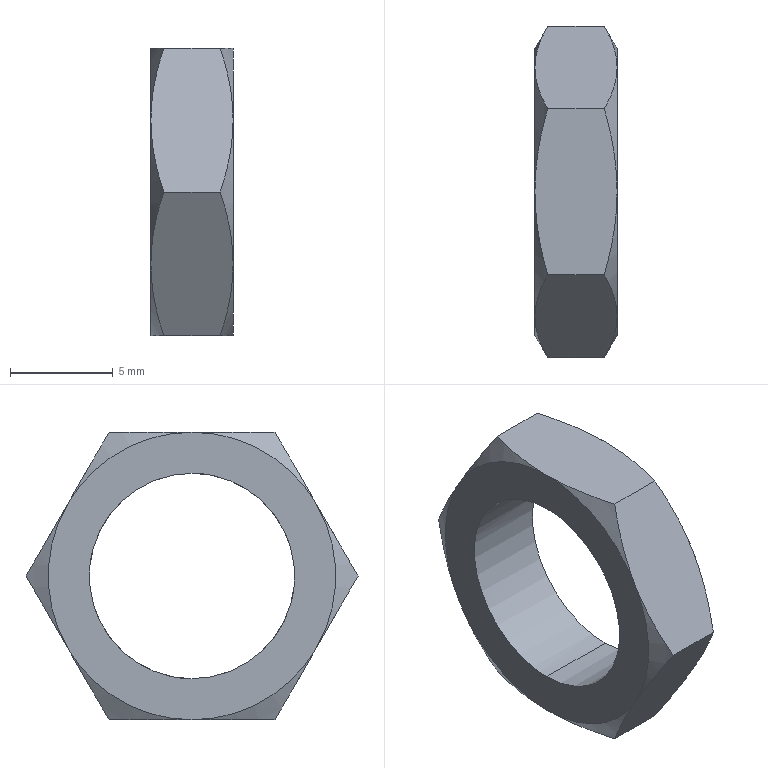Component | SolidWorks | 17268PB16x60SU(58)+(CS1-M-2)-1_1726816nut-1 | 1 solid | 22 faces | box 4 x 16.17 x 14 mm | volume 359 mm3 | cone 12 | plane 8 | cylinder 2 | commonest cylinder face diameters 10 x2
build123d program:
from build123d import *

# Parameters (mm, degrees)
CUT_EXTRUDE1_DEPTH               = 2
CUT_EXTRUDE1_DEPTH_BACK          = 2
SKETCH3_W                        = 28
SKETCH3_H                        = 28
THREAD_FIT_RELIEF_M10_DEPTH      = 12.416
THREAD_FIT_RELIEF_M10_DEPTH_BACK = 12.416
SKETCH1_R                        = 5


with BuildPart() as part:
    # Sketch1_2 → Revolve1 (revolve)
    with BuildSketch(Plane.XY, mode=Mode.PRIVATE) as revolve1_sk:
        Polygon((-2, 0), (-2, 7), (-1.192, 8.4), (1.192, 8.4), (2, 7), (2, 0), align=None)
    revolve(revolve1_sk.sketch.rotate(Axis((2, 0, 0), (-1, 0, 0)), 270), axis=Axis((2, 0, 0), (-1, 0, 0)))

    # Sketch2 → Cut-Revolve1 (revolve, cut)
    with BuildSketch(Plane.XY, mode=Mode.PRIVATE) as cut_revolve1_sk:
        Polygon((-2, 0), (-2, 5), (-1.188, 4.188), (1.188, 4.188), (2, 5), (2, 0), align=None)
    revolve(cut_revolve1_sk.sketch.rotate(Axis((2, 0, 0), (-1, 0, 0)), 270), axis=Axis((2, 0, 0), (-1, 0, 0)), mode=Mode.SUBTRACT)

    # Sketch3 → Cut-Extrude1 (cut, two sides: drawn at the far end of the back side and taken through both)
    with BuildSketch(Plane(origin=(0, 0, 0), x_dir=(0, 0, -1), z_dir=(1, 0, 0)).offset(-CUT_EXTRUDE1_DEPTH_BACK)):
        Rectangle(SKETCH3_W, SKETCH3_H)
        Polygon((-7, -4.041), (0, -8.083), (7, -4.041), (7, 4.041), (0, 8.083), (-7, 4.041), align=None, mode=Mode.SUBTRACT)
    extrude(amount=CUT_EXTRUDE1_DEPTH + CUT_EXTRUDE1_DEPTH_BACK, mode=Mode.SUBTRACT)

    # Sketch1 → Thread fit relief M10 (cut, two sides: drawn at the far end of the back side and taken through both)
    with BuildSketch(Plane.ZY.offset(2).offset(-THREAD_FIT_RELIEF_M10_DEPTH_BACK)):
        Circle(SKETCH1_R)
    extrude(amount=THREAD_FIT_RELIEF_M10_DEPTH + THREAD_FIT_RELIEF_M10_DEPTH_BACK, mode=Mode.SUBTRACT)


solid = part.part

# Placed as in the assembly
solid = solid.moved(Location((-73, -27.579, 21.5), (0, 0, 0)))
STEP:
#1=COLOUR_RGB('',0.7922,0.8196,0.9333);
#2=FILL_AREA_STYLE_COLOUR('',#1);
#3=FILL_AREA_STYLE('',(#2));
#4=SURFACE_STYLE_FILL_AREA(#3);
#5=SURFACE_SIDE_STYLE('',(#4));
#6=SURFACE_STYLE_USAGE(.BOTH.,#5);
#7=PRESENTATION_STYLE_ASSIGNMENT((#6));
#8=CARTESIAN_POINT('',(-2.795,-1.086,1.043));
#9=VERTEX_POINT('',#8);
#10=CARTESIAN_POINT('',(-2.795,-1.086,0.6496));
#11=VERTEX_POINT('',#10);
#12=CARTESIAN_POINT('',(-2.795,-1.086,0.8465));
#13=DIRECTION('',(-1.,0.,0.));
#14=DIRECTION('',(0.,0.,-1.));
#15=AXIS2_PLACEMENT_3D('',#12,#13,#14);
#16=CIRCLE('',#15,0.1969);
#17=EDGE_CURVE('',#9,#11,#16,.T.);
#18=ORIENTED_EDGE('',*,*,#17,.F.);
#19=CARTESIAN_POINT('',(-2.953,-1.086,1.043));
#20=VERTEX_POINT('',#19);
#21=CARTESIAN_POINT('',(-2.795,-1.086,1.043));
#22=DIRECTION('',(-1.,0.,0.));
#23=VECTOR('',#22,39.37);
#24=LINE('',#21,#23);
#25=EDGE_CURVE('',#9,#20,#24,.T.);
#26=ORIENTED_EDGE('',*,*,#25,.T.);
#27=CARTESIAN_POINT('',(-2.953,-1.086,0.6496));
#28=VERTEX_POINT('',#27);
#29=CARTESIAN_POINT('',(-2.953,-1.086,1.043));
#30=CARTESIAN_POINT('',(-2.953,-1.06,1.043));
#31=CARTESIAN_POINT('',(-2.953,-1.034,1.038));
#32=CARTESIAN_POINT('',(-2.953,-0.9867,1.018));
#33=CARTESIAN_POINT('',(-2.953,-0.9648,1.004));
#34=CARTESIAN_POINT('',(-2.953,-0.9284,0.9674));
#35=CARTESIAN_POINT('',(-2.953,-0.9138,0.9456));
#36=CARTESIAN_POINT('',(-2.953,-0.8941,0.898));
#37=CARTESIAN_POINT('',(-2.953,-0.8889,0.8722));
#38=CARTESIAN_POINT('',(-2.953,-0.8889,0.8207));
#39=CARTESIAN_POINT('',(-2.953,-0.8941,0.7949));
#40=CARTESIAN_POINT('',(-2.953,-0.9138,0.7473));
#41=CARTESIAN_POINT('',(-2.953,-0.9284,0.7255));
#42=CARTESIAN_POINT('',(-2.953,-0.9648,0.689));
#43=CARTESIAN_POINT('',(-2.953,-0.9867,0.6745));
#44=CARTESIAN_POINT('',(-2.953,-1.034,0.6547));
#45=CARTESIAN_POINT('',(-2.953,-1.06,0.6496));
#46=CARTESIAN_POINT('',(-2.953,-1.086,0.6496));
#47=B_SPLINE_CURVE_WITH_KNOTS('',3,(#29,#30,#31,#32,#33,#34,#35,#36,#37,#38,#39,#40,#41,#42,#43,#44,#45,#46),.UNSPECIFIED.,.F.,.F.,(4,2,2,2,2,2,2,2,4),(0.5,0.5625,0.625,0.6875,0.75,0.8125,0.875,0.9375,1.),.UNSPECIFIED.);
#48=EDGE_CURVE('',#20,#28,#47,.T.);
#49=ORIENTED_EDGE('',*,*,#48,.T.);
#50=CARTESIAN_POINT('',(-2.795,-1.086,0.6496));
#51=DIRECTION('',(-1.,0.,0.));
#52=VECTOR('',#51,39.37);
#53=LINE('',#50,#52);
#54=EDGE_CURVE('',#11,#28,#53,.T.);
#55=ORIENTED_EDGE('',*,*,#54,.F.);
#56=EDGE_LOOP('',(#18,#26,#49,#55));
#57=FACE_OUTER_BOUND('',#56,.T.);
#58=CARTESIAN_POINT('',(-2.795,-1.086,0.8465));
#59=DIRECTION('',(-1.,0.,0.));
#60=DIRECTION('',(0.,0.,-1.));
#61=AXIS2_PLACEMENT_3D('',#58,#59,#60);
#62=CYLINDRICAL_SURFACE('',#61,0.1969);
#63=ADVANCED_FACE('',(#57),#62,.F.);
#64=CARTESIAN_POINT('',(-2.928,-1.245,1.122));
#65=VERTEX_POINT('',#64);
#66=CARTESIAN_POINT('',(-2.953,-1.324,0.9843));
#67=VERTEX_POINT('',#66);
#68=CARTESIAN_POINT('',(-2.928,-1.245,1.122));
#69=CARTESIAN_POINT('',(-2.936,-1.258,1.1));
#70=CARTESIAN_POINT('',(-2.942,-1.271,1.077));
#71=CARTESIAN_POINT('',(-2.95,-1.298,1.031));
#72=CARTESIAN_POINT('',(-2.953,-1.311,1.008));
#73=CARTESIAN_POINT('',(-2.953,-1.324,0.9843));
#74=B_SPLINE_CURVE_WITH_KNOTS('',3,(#68,#69,#70,#71,#72,#73),.UNSPECIFIED.,.F.,.F.,(4,2,4),(0.00000024,0.002045,0.00409),.UNSPECIFIED.);
#75=EDGE_CURVE('',#65,#67,#74,.T.);
#76=ORIENTED_EDGE('',*,*,#75,.F.);
#77=CARTESIAN_POINT('',(-2.953,-1.086,1.122));
#78=VERTEX_POINT('',#77);
#79=CARTESIAN_POINT('',(-2.953,-1.086,1.122));
#80=CARTESIAN_POINT('',(-2.953,-1.113,1.122));
#81=CARTESIAN_POINT('',(-2.95,-1.14,1.122));
#82=CARTESIAN_POINT('',(-2.942,-1.193,1.122));
#83=CARTESIAN_POINT('',(-2.936,-1.219,1.122));
#84=CARTESIAN_POINT('',(-2.928,-1.245,1.122));
#85=B_SPLINE_CURVE_WITH_KNOTS('',3,(#79,#80,#81,#82,#83,#84),.UNSPECIFIED.,.F.,.F.,(4,2,4),(0.01133,0.01337,0.01542),.UNSPECIFIED.);
#86=EDGE_CURVE('',#78,#65,#85,.T.);
#87=ORIENTED_EDGE('',*,*,#86,.F.);
#88=CARTESIAN_POINT('',(-2.953,-1.086,0.8465));
#89=DIRECTION('',(-1.,0.,0.));
#90=DIRECTION('',(0.,0.,-1.));
#91=AXIS2_PLACEMENT_3D('',#88,#89,#90);
#92=CIRCLE('',#91,0.2756);
#93=EDGE_CURVE('',#67,#78,#92,.T.);
#94=ORIENTED_EDGE('',*,*,#93,.F.);
#95=EDGE_LOOP('',(#76,#87,#94));
#96=FACE_OUTER_BOUND('',#95,.T.);
#97=CARTESIAN_POINT('',(-2.921,-1.086,0.8465));
#98=DIRECTION('',(1.,-0.,-0.));
#99=DIRECTION('',(0.,0.,1.));
#100=AXIS2_PLACEMENT_3D('',#97,#98,#99);
#101=CONICAL_SURFACE('',#100,0.3307,1.047);
#102=ADVANCED_FACE('',(#96),#101,.T.);
#103=CARTESIAN_POINT('',(-2.928,-1.404,0.8465));
#104=VERTEX_POINT('',#103);
#105=CARTESIAN_POINT('',(-2.953,-1.324,0.9843));
#106=CARTESIAN_POINT('',(-2.953,-1.331,0.9726));
#107=CARTESIAN_POINT('',(-2.952,-1.338,0.9608));
#108=CARTESIAN_POINT('',(-2.95,-1.351,0.9376));
#109=CARTESIAN_POINT('',(-2.948,-1.358,0.926));
#110=CARTESIAN_POINT('',(-2.942,-1.378,0.8916));
#111=CARTESIAN_POINT('',(-2.936,-1.391,0.8689));
#112=CARTESIAN_POINT('',(-2.928,-1.404,0.8465));
#113=B_SPLINE_CURVE_WITH_KNOTS('',3,(#105,#106,#107,#108,#109,#110,#111,#112),.UNSPECIFIED.,.F.,.F.,(4,2,2,4),(0.00409,0.005108,0.006127,0.008164),.UNSPECIFIED.);
#114=EDGE_CURVE('',#67,#104,#113,.T.);
#115=ORIENTED_EDGE('',*,*,#114,.F.);
#116=CARTESIAN_POINT('',(-2.953,-1.324,0.7087));
#117=VERTEX_POINT('',#116);
#118=CARTESIAN_POINT('',(-2.953,-1.086,0.8465));
#119=DIRECTION('',(-1.,0.,0.));
#120=DIRECTION('',(0.,0.,-1.));
#121=AXIS2_PLACEMENT_3D('',#118,#119,#120);
#122=CIRCLE('',#121,0.2756);
#123=EDGE_CURVE('',#117,#67,#122,.T.);
#124=ORIENTED_EDGE('',*,*,#123,.F.);
#125=CARTESIAN_POINT('',(-2.928,-1.404,0.8465));
#126=CARTESIAN_POINT('',(-2.936,-1.391,0.8239));
#127=CARTESIAN_POINT('',(-2.942,-1.378,0.8012));
#128=CARTESIAN_POINT('',(-2.95,-1.351,0.7553));
#129=CARTESIAN_POINT('',(-2.953,-1.338,0.7321));
#130=CARTESIAN_POINT('',(-2.953,-1.324,0.7087));
#131=B_SPLINE_CURVE_WITH_KNOTS('',3,(#125,#126,#127,#128,#129,#130),.UNSPECIFIED.,.F.,.F.,(4,2,4),(0.00000024,0.002045,0.00409),.UNSPECIFIED.);
#132=EDGE_CURVE('',#104,#117,#131,.T.);
#133=ORIENTED_EDGE('',*,*,#132,.F.);
#134=EDGE_LOOP('',(#115,#124,#133));
#135=FACE_OUTER_BOUND('',#134,.T.);
#136=CARTESIAN_POINT('',(-2.921,-1.086,0.8465));
#137=DIRECTION('',(1.,-0.,-0.));
#138=DIRECTION('',(0.,0.,1.));
#139=AXIS2_PLACEMENT_3D('',#136,#137,#138);
#140=CONICAL_SURFACE('',#139,0.3307,1.047);
#141=ADVANCED_FACE('',(#135),#140,.T.);
#142=CARTESIAN_POINT('',(-2.928,-1.245,0.5709));
#143=VERTEX_POINT('',#142);
#144=CARTESIAN_POINT('',(-2.953,-1.324,0.7087));
#145=CARTESIAN_POINT('',(-2.953,-1.318,0.697));
#146=CARTESIAN_POINT('',(-2.952,-1.311,0.6852));
#147=CARTESIAN_POINT('',(-2.95,-1.298,0.662));
#148=CARTESIAN_POINT('',(-2.948,-1.291,0.6504));
#149=CARTESIAN_POINT('',(-2.942,-1.271,0.616));
#150=CARTESIAN_POINT('',(-2.936,-1.258,0.5934));
#151=CARTESIAN_POINT('',(-2.928,-1.245,0.5709));
#152=B_SPLINE_CURVE_WITH_KNOTS('',3,(#144,#145,#146,#147,#148,#149,#150,#151),.UNSPECIFIED.,.F.,.F.,(4,2,2,4),(0.00409,0.005108,0.006127,0.008164),.UNSPECIFIED.);
#153=EDGE_CURVE('',#117,#143,#152,.T.);
#154=ORIENTED_EDGE('',*,*,#153,.F.);
#155=CARTESIAN_POINT('',(-2.953,-1.086,0.5709));
#156=VERTEX_POINT('',#155);
#157=CARTESIAN_POINT('',(-2.953,-1.086,0.8465));
#158=DIRECTION('',(-1.,0.,0.));
#159=DIRECTION('',(0.,0.,-1.));
#160=AXIS2_PLACEMENT_3D('',#157,#158,#159);
#161=CIRCLE('',#160,0.2756);
#162=EDGE_CURVE('',#156,#117,#161,.T.);
#163=ORIENTED_EDGE('',*,*,#162,.F.);
#164=CARTESIAN_POINT('',(-2.928,-1.245,0.5709));
#165=CARTESIAN_POINT('',(-2.936,-1.219,0.5709));
#166=CARTESIAN_POINT('',(-2.942,-1.193,0.5709));
#167=CARTESIAN_POINT('',(-2.95,-1.14,0.5709));
#168=CARTESIAN_POINT('',(-2.953,-1.113,0.5709));
#169=CARTESIAN_POINT('',(-2.953,-1.086,0.5709));
#170=B_SPLINE_CURVE_WITH_KNOTS('',3,(#164,#165,#166,#167,#168,#169),.UNSPECIFIED.,.F.,.F.,(4,2,4),(0.01774,0.01979,0.02184),.UNSPECIFIED.);
#171=EDGE_CURVE('',#143,#156,#170,.T.);
#172=ORIENTED_EDGE('',*,*,#171,.F.);
#173=EDGE_LOOP('',(#154,#163,#172));
#174=FACE_OUTER_BOUND('',#173,.T.);
#175=CARTESIAN_POINT('',(-2.921,-1.086,0.8465));
#176=DIRECTION('',(1.,-0.,-0.));
#177=DIRECTION('',(0.,0.,1.));
#178=AXIS2_PLACEMENT_3D('',#175,#176,#177);
#179=CONICAL_SURFACE('',#178,0.3307,1.047);
#180=ADVANCED_FACE('',(#174),#179,.T.);
#181=CARTESIAN_POINT('',(-2.928,-0.9267,1.122));
#182=VERTEX_POINT('',#181);
#183=CARTESIAN_POINT('',(-2.928,-0.9267,1.122));
#184=CARTESIAN_POINT('',(-2.936,-0.9526,1.122));
#185=CARTESIAN_POINT('',(-2.942,-0.9791,1.122));
#186=CARTESIAN_POINT('',(-2.95,-1.032,1.122));
#187=CARTESIAN_POINT('',(-2.953,-1.059,1.122));
#188=CARTESIAN_POINT('',(-2.953,-1.086,1.122));
#189=B_SPLINE_CURVE_WITH_KNOTS('',3,(#183,#184,#185,#186,#187,#188),.UNSPECIFIED.,.F.,.F.,(4,2,4),(0.007239,0.009283,0.01133),.UNSPECIFIED.);
#190=EDGE_CURVE('',#182,#78,#189,.T.);
#191=ORIENTED_EDGE('',*,*,#190,.F.);
#192=CARTESIAN_POINT('',(-2.953,-0.8471,0.9843));
#193=VERTEX_POINT('',#192);
#194=CARTESIAN_POINT('',(-2.953,-0.8471,0.9843));
#195=CARTESIAN_POINT('',(-2.953,-0.8539,0.9959));
#196=CARTESIAN_POINT('',(-2.952,-0.8607,1.008));
#197=CARTESIAN_POINT('',(-2.95,-0.8741,1.031));
#198=CARTESIAN_POINT('',(-2.948,-0.8807,1.042));
#199=CARTESIAN_POINT('',(-2.942,-0.9006,1.077));
#200=CARTESIAN_POINT('',(-2.936,-0.9137,1.1));
#201=CARTESIAN_POINT('',(-2.928,-0.9267,1.122));
#202=B_SPLINE_CURVE_WITH_KNOTS('',3,(#194,#195,#196,#197,#198,#199,#200,#201),.UNSPECIFIED.,.F.,.F.,(4,2,2,4),(0.00409,0.005108,0.006127,0.008164),.UNSPECIFIED.);
#203=EDGE_CURVE('',#193,#182,#202,.T.);
#204=ORIENTED_EDGE('',*,*,#203,.F.);
#205=CARTESIAN_POINT('',(-2.953,-1.086,0.8465));
#206=DIRECTION('',(-1.,0.,0.));
#207=DIRECTION('',(0.,0.,-1.));
#208=AXIS2_PLACEMENT_3D('',#205,#206,#207);
#209=CIRCLE('',#208,0.2756);
#210=EDGE_CURVE('',#78,#193,#209,.T.);
#211=ORIENTED_EDGE('',*,*,#210,.F.);
#212=EDGE_LOOP('',(#191,#204,#211));
#213=FACE_OUTER_BOUND('',#212,.T.);
#214=CARTESIAN_POINT('',(-2.921,-1.086,0.8465));
#215=DIRECTION('',(1.,-0.,-0.));
#216=DIRECTION('',(0.,0.,1.));
#217=AXIS2_PLACEMENT_3D('',#214,#215,#216);
#218=CONICAL_SURFACE('',#217,0.3307,1.047);
#219=ADVANCED_FACE('',(#213),#218,.T.);
#220=CARTESIAN_POINT('',(-2.928,-0.9267,0.5709));
#221=VERTEX_POINT('',#220);
#222=CARTESIAN_POINT('',(-2.953,-1.086,0.5709));
#223=CARTESIAN_POINT('',(-2.953,-1.059,0.5709));
#224=CARTESIAN_POINT('',(-2.95,-1.032,0.5709));
#225=CARTESIAN_POINT('',(-2.942,-0.9791,0.5709));
#226=CARTESIAN_POINT('',(-2.936,-0.9526,0.5709));
#227=CARTESIAN_POINT('',(-2.928,-0.9267,0.5709));
#228=B_SPLINE_CURVE_WITH_KNOTS('',3,(#222,#223,#224,#225,#226,#227),.UNSPECIFIED.,.F.,.F.,(4,2,4),(0.02184,0.02388,0.02593),.UNSPECIFIED.);
#229=EDGE_CURVE('',#156,#221,#228,.T.);
#230=ORIENTED_EDGE('',*,*,#229,.F.);
#231=CARTESIAN_POINT('',(-2.953,-0.8471,0.7087));
#232=VERTEX_POINT('',#231);
#233=CARTESIAN_POINT('',(-2.953,-1.086,0.8465));
#234=DIRECTION('',(-1.,0.,0.));
#235=DIRECTION('',(0.,0.,-1.));
#236=AXIS2_PLACEMENT_3D('',#233,#234,#235);
#237=CIRCLE('',#236,0.2756);
#238=EDGE_CURVE('',#232,#156,#237,.T.);
#239=ORIENTED_EDGE('',*,*,#238,.F.);
#240=CARTESIAN_POINT('',(-2.928,-0.9267,0.5709));
#241=CARTESIAN_POINT('',(-2.936,-0.9137,0.5934));
#242=CARTESIAN_POINT('',(-2.942,-0.9006,0.6161));
#243=CARTESIAN_POINT('',(-2.95,-0.8741,0.662));
#244=CARTESIAN_POINT('',(-2.953,-0.8607,0.6852));
#245=CARTESIAN_POINT('',(-2.953,-0.8471,0.7087));
#246=B_SPLINE_CURVE_WITH_KNOTS('',3,(#240,#241,#242,#243,#244,#245),.UNSPECIFIED.,.F.,.F.,(4,2,4),(0.00000024,0.002045,0.00409),.UNSPECIFIED.);
#247=EDGE_CURVE('',#221,#232,#246,.T.);
#248=ORIENTED_EDGE('',*,*,#247,.F.);
#249=EDGE_LOOP('',(#230,#239,#248));
#250=FACE_OUTER_BOUND('',#249,.T.);
#251=CARTESIAN_POINT('',(-2.921,-1.086,0.8465));
#252=DIRECTION('',(1.,-0.,-0.));
#253=DIRECTION('',(0.,0.,1.));
#254=AXIS2_PLACEMENT_3D('',#251,#252,#253);
#255=CONICAL_SURFACE('',#254,0.3307,1.047);
#256=ADVANCED_FACE('',(#250),#255,.T.);
#257=CARTESIAN_POINT('',(-2.928,-0.7676,0.8465));
#258=VERTEX_POINT('',#257);
#259=CARTESIAN_POINT('',(-2.928,-0.7676,0.8465));
#260=CARTESIAN_POINT('',(-2.936,-0.7806,0.869));
#261=CARTESIAN_POINT('',(-2.942,-0.7937,0.8917));
#262=CARTESIAN_POINT('',(-2.95,-0.8202,0.9376));
#263=CARTESIAN_POINT('',(-2.953,-0.8336,0.9608));
#264=CARTESIAN_POINT('',(-2.953,-0.8471,0.9843));
#265=B_SPLINE_CURVE_WITH_KNOTS('',3,(#259,#260,#261,#262,#263,#264),.UNSPECIFIED.,.F.,.F.,(4,2,4),(0.00000024,0.002045,0.00409),.UNSPECIFIED.);
#266=EDGE_CURVE('',#258,#193,#265,.T.);
#267=ORIENTED_EDGE('',*,*,#266,.F.);
#268=CARTESIAN_POINT('',(-2.953,-0.8471,0.7087));
#269=CARTESIAN_POINT('',(-2.953,-0.8404,0.7204));
#270=CARTESIAN_POINT('',(-2.952,-0.8336,0.7321));
#271=CARTESIAN_POINT('',(-2.95,-0.8202,0.7553));
#272=CARTESIAN_POINT('',(-2.948,-0.8135,0.7669));
#273=CARTESIAN_POINT('',(-2.942,-0.7936,0.8013));
#274=CARTESIAN_POINT('',(-2.936,-0.7806,0.824));
#275=CARTESIAN_POINT('',(-2.928,-0.7676,0.8465));
#276=B_SPLINE_CURVE_WITH_KNOTS('',3,(#268,#269,#270,#271,#272,#273,#274,#275),.UNSPECIFIED.,.F.,.F.,(4,2,2,4),(0.00409,0.005108,0.006127,0.008164),.UNSPECIFIED.);
#277=EDGE_CURVE('',#232,#258,#276,.T.);
#278=ORIENTED_EDGE('',*,*,#277,.F.);
#279=CARTESIAN_POINT('',(-2.953,-1.086,0.8465));
#280=DIRECTION('',(-1.,0.,0.));
#281=DIRECTION('',(0.,0.,-1.));
#282=AXIS2_PLACEMENT_3D('',#279,#280,#281);
#283=CIRCLE('',#282,0.2756);
#284=EDGE_CURVE('',#193,#232,#283,.T.);
#285=ORIENTED_EDGE('',*,*,#284,.F.);
#286=EDGE_LOOP('',(#267,#278,#285));
#287=FACE_OUTER_BOUND('',#286,.T.);
#288=CARTESIAN_POINT('',(-2.921,-1.086,0.8465));
#289=DIRECTION('',(1.,-0.,-0.));
#290=DIRECTION('',(0.,0.,1.));
#291=AXIS2_PLACEMENT_3D('',#288,#289,#290);
#292=CONICAL_SURFACE('',#291,0.3307,1.047);
#293=ADVANCED_FACE('',(#287),#292,.T.);
#294=CARTESIAN_POINT('',(-2.82,-0.9267,0.5709));
#295=VERTEX_POINT('',#294);
#296=CARTESIAN_POINT('',(-2.795,-1.086,0.5709));
#297=VERTEX_POINT('',#296);
#298=CARTESIAN_POINT('',(-2.82,-0.9267,0.5709));
#299=CARTESIAN_POINT('',(-2.812,-0.9526,0.5709));
#300=CARTESIAN_POINT('',(-2.806,-0.9791,0.5709));
#301=CARTESIAN_POINT('',(-2.798,-1.032,0.5709));
#302=CARTESIAN_POINT('',(-2.795,-1.059,0.5709));
#303=CARTESIAN_POINT('',(-2.795,-1.086,0.5709));
#304=B_SPLINE_CURVE_WITH_KNOTS('',3,(#298,#299,#300,#301,#302,#303),.UNSPECIFIED.,.F.,.F.,(4,2,4),(0.007239,0.009283,0.01133),.UNSPECIFIED.);
#305=EDGE_CURVE('',#295,#297,#304,.T.);
#306=ORIENTED_EDGE('',*,*,#305,.F.);
#307=CARTESIAN_POINT('',(-2.795,-0.8471,0.7087));
#308=VERTEX_POINT('',#307);
#309=CARTESIAN_POINT('',(-2.795,-0.8471,0.7087));
#310=CARTESIAN_POINT('',(-2.795,-0.8539,0.697));
#311=CARTESIAN_POINT('',(-2.796,-0.8607,0.6852));
#312=CARTESIAN_POINT('',(-2.798,-0.8741,0.662));
#313=CARTESIAN_POINT('',(-2.8,-0.8807,0.6504));
#314=CARTESIAN_POINT('',(-2.806,-0.9006,0.616));
#315=CARTESIAN_POINT('',(-2.812,-0.9137,0.5934));
#316=CARTESIAN_POINT('',(-2.82,-0.9267,0.5709));
#317=B_SPLINE_CURVE_WITH_KNOTS('',3,(#309,#310,#311,#312,#313,#314,#315,#316),.UNSPECIFIED.,.F.,.F.,(4,2,2,4),(0.00409,0.005108,0.006127,0.008164),.UNSPECIFIED.);
#318=EDGE_CURVE('',#308,#295,#317,.T.);
#319=ORIENTED_EDGE('',*,*,#318,.F.);
#320=CARTESIAN_POINT('',(-2.795,-1.086,0.8465));
#321=DIRECTION('',(-1.,0.,0.));
#322=DIRECTION('',(0.,0.,-1.));
#323=AXIS2_PLACEMENT_3D('',#320,#321,#322);
#324=CIRCLE('',#323,0.2756);
#325=EDGE_CURVE('',#308,#297,#324,.T.);
#326=ORIENTED_EDGE('',*,*,#325,.T.);
#327=EDGE_LOOP('',(#306,#319,#326));
#328=FACE_OUTER_BOUND('',#327,.T.);
#329=CARTESIAN_POINT('',(-2.795,-1.086,0.8465));
#330=DIRECTION('',(-1.,0.,0.));
#331=DIRECTION('',(0.,0.,-1.));
#332=AXIS2_PLACEMENT_3D('',#329,#330,#331);
#333=CONICAL_SURFACE('',#332,0.2756,1.047);
#334=ADVANCED_FACE('',(#328),#333,.T.);
#335=CARTESIAN_POINT('',(-2.82,-1.245,0.5709));
#336=VERTEX_POINT('',#335);
#337=CARTESIAN_POINT('',(-2.795,-1.086,0.5709));
#338=CARTESIAN_POINT('',(-2.795,-1.113,0.5709));
#339=CARTESIAN_POINT('',(-2.798,-1.14,0.5709));
#340=CARTESIAN_POINT('',(-2.806,-1.193,0.5709));
#341=CARTESIAN_POINT('',(-2.812,-1.219,0.5709));
#342=CARTESIAN_POINT('',(-2.82,-1.245,0.5709));
#343=B_SPLINE_CURVE_WITH_KNOTS('',3,(#337,#338,#339,#340,#341,#342),.UNSPECIFIED.,.F.,.F.,(4,2,4),(0.01133,0.01337,0.01542),.UNSPECIFIED.);
#344=EDGE_CURVE('',#297,#336,#343,.T.);
#345=ORIENTED_EDGE('',*,*,#344,.F.);
#346=CARTESIAN_POINT('',(-2.795,-1.324,0.7087));
#347=VERTEX_POINT('',#346);
#348=CARTESIAN_POINT('',(-2.795,-1.086,0.8465));
#349=DIRECTION('',(-1.,0.,0.));
#350=DIRECTION('',(0.,0.,-1.));
#351=AXIS2_PLACEMENT_3D('',#348,#349,#350);
#352=CIRCLE('',#351,0.2756);
#353=EDGE_CURVE('',#297,#347,#352,.T.);
#354=ORIENTED_EDGE('',*,*,#353,.T.);
#355=CARTESIAN_POINT('',(-2.82,-1.245,0.5709));
#356=CARTESIAN_POINT('',(-2.812,-1.258,0.5934));
#357=CARTESIAN_POINT('',(-2.806,-1.271,0.6161));
#358=CARTESIAN_POINT('',(-2.798,-1.298,0.662));
#359=CARTESIAN_POINT('',(-2.795,-1.311,0.6852));
#360=CARTESIAN_POINT('',(-2.795,-1.324,0.7087));
#361=B_SPLINE_CURVE_WITH_KNOTS('',3,(#355,#356,#357,#358,#359,#360),.UNSPECIFIED.,.F.,.F.,(4,2,4),(0.00000024,0.002045,0.00409),.UNSPECIFIED.);
#362=EDGE_CURVE('',#336,#347,#361,.T.);
#363=ORIENTED_EDGE('',*,*,#362,.F.);
#364=EDGE_LOOP('',(#345,#354,#363));
#365=FACE_OUTER_BOUND('',#364,.T.);
#366=CARTESIAN_POINT('',(-2.795,-1.086,0.8465));
#367=DIRECTION('',(-1.,0.,0.));
#368=DIRECTION('',(0.,0.,-1.));
#369=AXIS2_PLACEMENT_3D('',#366,#367,#368);
#370=CONICAL_SURFACE('',#369,0.2756,1.047);
#371=ADVANCED_FACE('',(#365),#370,.T.);
#372=CARTESIAN_POINT('',(-2.82,-1.404,0.8465));
#373=VERTEX_POINT('',#372);
#374=CARTESIAN_POINT('',(-2.795,-1.324,0.7087));
#375=CARTESIAN_POINT('',(-2.795,-1.331,0.7204));
#376=CARTESIAN_POINT('',(-2.796,-1.338,0.7321));
#377=CARTESIAN_POINT('',(-2.798,-1.351,0.7553));
#378=CARTESIAN_POINT('',(-2.8,-1.358,0.7669));
#379=CARTESIAN_POINT('',(-2.806,-1.378,0.8013));
#380=CARTESIAN_POINT('',(-2.812,-1.391,0.824));
#381=CARTESIAN_POINT('',(-2.82,-1.404,0.8465));
#382=B_SPLINE_CURVE_WITH_KNOTS('',3,(#374,#375,#376,#377,#378,#379,#380,#381),.UNSPECIFIED.,.F.,.F.,(4,2,2,4),(0.00409,0.005108,0.006127,0.008164),.UNSPECIFIED.);
#383=EDGE_CURVE('',#347,#373,#382,.T.);
#384=ORIENTED_EDGE('',*,*,#383,.F.);
#385=CARTESIAN_POINT('',(-2.795,-1.324,0.9843));
#386=VERTEX_POINT('',#385);
#387=CARTESIAN_POINT('',(-2.795,-1.086,0.8465));
#388=DIRECTION('',(-1.,0.,0.));
#389=DIRECTION('',(0.,0.,-1.));
#390=AXIS2_PLACEMENT_3D('',#387,#388,#389);
#391=CIRCLE('',#390,0.2756);
#392=EDGE_CURVE('',#347,#386,#391,.T.);
#393=ORIENTED_EDGE('',*,*,#392,.T.);
#394=CARTESIAN_POINT('',(-2.82,-1.404,0.8465));
#395=CARTESIAN_POINT('',(-2.812,-1.391,0.869));
#396=CARTESIAN_POINT('',(-2.806,-1.378,0.8917));
#397=CARTESIAN_POINT('',(-2.798,-1.351,0.9376));
#398=CARTESIAN_POINT('',(-2.795,-1.338,0.9608));
#399=CARTESIAN_POINT('',(-2.795,-1.324,0.9843));
#400=B_SPLINE_CURVE_WITH_KNOTS('',3,(#394,#395,#396,#397,#398,#399),.UNSPECIFIED.,.F.,.F.,(4,2,4),(0.00000024,0.002045,0.00409),.UNSPECIFIED.);
#401=EDGE_CURVE('',#373,#386,#400,.T.);
#402=ORIENTED_EDGE('',*,*,#401,.F.);
#403=EDGE_LOOP('',(#384,#393,#402));
#404=FACE_OUTER_BOUND('',#403,.T.);
#405=CARTESIAN_POINT('',(-2.795,-1.086,0.8465));
#406=DIRECTION('',(-1.,0.,0.));
#407=DIRECTION('',(0.,0.,-1.));
#408=AXIS2_PLACEMENT_3D('',#405,#406,#407);
#409=CONICAL_SURFACE('',#408,0.2756,1.047);
#410=ADVANCED_FACE('',(#404),#409,.T.);
#411=CARTESIAN_POINT('',(-2.82,-1.245,1.122));
#412=VERTEX_POINT('',#411);
#413=CARTESIAN_POINT('',(-2.795,-1.324,0.9843));
#414=CARTESIAN_POINT('',(-2.795,-1.318,0.9959));
#415=CARTESIAN_POINT('',(-2.796,-1.311,1.008));
#416=CARTESIAN_POINT('',(-2.798,-1.298,1.031));
#417=CARTESIAN_POINT('',(-2.8,-1.291,1.042));
#418=CARTESIAN_POINT('',(-2.806,-1.271,1.077));
#419=CARTESIAN_POINT('',(-2.812,-1.258,1.1));
#420=CARTESIAN_POINT('',(-2.82,-1.245,1.122));
#421=B_SPLINE_CURVE_WITH_KNOTS('',3,(#413,#414,#415,#416,#417,#418,#419,#420),.UNSPECIFIED.,.F.,.F.,(4,2,2,4),(0.00409,0.005108,0.006127,0.008164),.UNSPECIFIED.);
#422=EDGE_CURVE('',#386,#412,#421,.T.);
#423=ORIENTED_EDGE('',*,*,#422,.F.);
#424=CARTESIAN_POINT('',(-2.795,-1.086,1.122));
#425=VERTEX_POINT('',#424);
#426=CARTESIAN_POINT('',(-2.795,-1.086,0.8465));
#427=DIRECTION('',(-1.,0.,0.));
#428=DIRECTION('',(0.,0.,-1.));
#429=AXIS2_PLACEMENT_3D('',#426,#427,#428);
#430=CIRCLE('',#429,0.2756);
#431=EDGE_CURVE('',#386,#425,#430,.T.);
#432=ORIENTED_EDGE('',*,*,#431,.T.);
#433=CARTESIAN_POINT('',(-2.82,-1.245,1.122));
#434=CARTESIAN_POINT('',(-2.812,-1.219,1.122));
#435=CARTESIAN_POINT('',(-2.806,-1.193,1.122));
#436=CARTESIAN_POINT('',(-2.798,-1.14,1.122));
#437=CARTESIAN_POINT('',(-2.795,-1.113,1.122));
#438=CARTESIAN_POINT('',(-2.795,-1.086,1.122));
#439=B_SPLINE_CURVE_WITH_KNOTS('',3,(#433,#434,#435,#436,#437,#438),.UNSPECIFIED.,.F.,.F.,(4,2,4),(0.01774,0.01979,0.02184),.UNSPECIFIED.);
#440=EDGE_CURVE('',#412,#425,#439,.T.);
#441=ORIENTED_EDGE('',*,*,#440,.F.);
#442=EDGE_LOOP('',(#423,#432,#441));
#443=FACE_OUTER_BOUND('',#442,.T.);
#444=CARTESIAN_POINT('',(-2.795,-1.086,0.8465));
#445=DIRECTION('',(-1.,0.,0.));
#446=DIRECTION('',(0.,0.,-1.));
#447=AXIS2_PLACEMENT_3D('',#444,#445,#446);
#448=CONICAL_SURFACE('',#447,0.2756,1.047);
#449=ADVANCED_FACE('',(#443),#448,.T.);
#450=CARTESIAN_POINT('',(-2.82,-0.9267,1.122));
#451=VERTEX_POINT('',#450);
#452=CARTESIAN_POINT('',(-2.795,-1.086,1.122));
#453=CARTESIAN_POINT('',(-2.795,-1.059,1.122));
#454=CARTESIAN_POINT('',(-2.798,-1.032,1.122));
#455=CARTESIAN_POINT('',(-2.806,-0.9791,1.122));
#456=CARTESIAN_POINT('',(-2.812,-0.9526,1.122));
#457=CARTESIAN_POINT('',(-2.82,-0.9267,1.122));
#458=B_SPLINE_CURVE_WITH_KNOTS('',3,(#452,#453,#454,#455,#456,#457),.UNSPECIFIED.,.F.,.F.,(4,2,4),(0.02184,0.02388,0.02593),.UNSPECIFIED.);
#459=EDGE_CURVE('',#425,#451,#458,.T.);
#460=ORIENTED_EDGE('',*,*,#459,.F.);
#461=CARTESIAN_POINT('',(-2.795,-0.8471,0.9843));
#462=VERTEX_POINT('',#461);
#463=CARTESIAN_POINT('',(-2.795,-1.086,0.8465));
#464=DIRECTION('',(-1.,0.,0.));
#465=DIRECTION('',(0.,0.,-1.));
#466=AXIS2_PLACEMENT_3D('',#463,#464,#465);
#467=CIRCLE('',#466,0.2756);
#468=EDGE_CURVE('',#425,#462,#467,.T.);
#469=ORIENTED_EDGE('',*,*,#468,.T.);
#470=CARTESIAN_POINT('',(-2.82,-0.9267,1.122));
#471=CARTESIAN_POINT('',(-2.812,-0.9137,1.1));
#472=CARTESIAN_POINT('',(-2.806,-0.9006,1.077));
#473=CARTESIAN_POINT('',(-2.798,-0.8741,1.031));
#474=CARTESIAN_POINT('',(-2.795,-0.8607,1.008));
#475=CARTESIAN_POINT('',(-2.795,-0.8471,0.9843));
#476=B_SPLINE_CURVE_WITH_KNOTS('',3,(#470,#471,#472,#473,#474,#475),.UNSPECIFIED.,.F.,.F.,(4,2,4),(0.00000024,0.002045,0.00409),.UNSPECIFIED.);
#477=EDGE_CURVE('',#451,#462,#476,.T.);
#478=ORIENTED_EDGE('',*,*,#477,.F.);
#479=EDGE_LOOP('',(#460,#469,#478));
#480=FACE_OUTER_BOUND('',#479,.T.);
#481=CARTESIAN_POINT('',(-2.795,-1.086,0.8465));
#482=DIRECTION('',(-1.,0.,0.));
#483=DIRECTION('',(0.,0.,-1.));
#484=AXIS2_PLACEMENT_3D('',#481,#482,#483);
#485=CONICAL_SURFACE('',#484,0.2756,1.047);
#486=ADVANCED_FACE('',(#480),#485,.T.);
#487=CARTESIAN_POINT('',(-2.82,-0.7676,0.8465));
#488=VERTEX_POINT('',#487);
#489=CARTESIAN_POINT('',(-2.795,-0.8471,0.9843));
#490=CARTESIAN_POINT('',(-2.795,-0.8404,0.9726));
#491=CARTESIAN_POINT('',(-2.796,-0.8336,0.9608));
#492=CARTESIAN_POINT('',(-2.798,-0.8202,0.9376));
#493=CARTESIAN_POINT('',(-2.8,-0.8135,0.926));
#494=CARTESIAN_POINT('',(-2.806,-0.7936,0.8916));
#495=CARTESIAN_POINT('',(-2.812,-0.7806,0.8689));
#496=CARTESIAN_POINT('',(-2.82,-0.7676,0.8465));
#497=B_SPLINE_CURVE_WITH_KNOTS('',3,(#489,#490,#491,#492,#493,#494,#495,#496),.UNSPECIFIED.,.F.,.F.,(4,2,2,4),(0.00409,0.005108,0.006127,0.008164),.UNSPECIFIED.);
#498=EDGE_CURVE('',#462,#488,#497,.T.);
#499=ORIENTED_EDGE('',*,*,#498,.F.);
#500=CARTESIAN_POINT('',(-2.795,-1.086,0.8465));
#501=DIRECTION('',(-1.,0.,0.));
#502=DIRECTION('',(0.,0.,-1.));
#503=AXIS2_PLACEMENT_3D('',#500,#501,#502);
#504=CIRCLE('',#503,0.2756);
#505=EDGE_CURVE('',#462,#308,#504,.T.);
#506=ORIENTED_EDGE('',*,*,#505,.T.);
#507=CARTESIAN_POINT('',(-2.82,-0.7676,0.8465));
#508=CARTESIAN_POINT('',(-2.812,-0.7806,0.8239));
#509=CARTESIAN_POINT('',(-2.806,-0.7937,0.8012));
#510=CARTESIAN_POINT('',(-2.798,-0.8202,0.7553));
#511=CARTESIAN_POINT('',(-2.795,-0.8336,0.7321));
#512=CARTESIAN_POINT('',(-2.795,-0.8471,0.7087));
#513=B_SPLINE_CURVE_WITH_KNOTS('',3,(#507,#508,#509,#510,#511,#512),.UNSPECIFIED.,.F.,.F.,(4,2,4),(0.00000024,0.002045,0.00409),.UNSPECIFIED.);
#514=EDGE_CURVE('',#488,#308,#513,.T.);
#515=ORIENTED_EDGE('',*,*,#514,.F.);
#516=EDGE_LOOP('',(#499,#506,#515));
#517=FACE_OUTER_BOUND('',#516,.T.);
#518=CARTESIAN_POINT('',(-2.795,-1.086,0.8465));
#519=DIRECTION('',(-1.,0.,0.));
#520=DIRECTION('',(0.,0.,-1.));
#521=AXIS2_PLACEMENT_3D('',#518,#519,#520);
#522=CONICAL_SURFACE('',#521,0.2756,1.047);
#523=ADVANCED_FACE('',(#517),#522,.T.);
#524=CARTESIAN_POINT('',(-2.953,-1.086,0.6496));
#525=CARTESIAN_POINT('',(-2.953,-1.112,0.6496));
#526=CARTESIAN_POINT('',(-2.953,-1.137,0.6547));
#527=CARTESIAN_POINT('',(-2.953,-1.185,0.6745));
#528=CARTESIAN_POINT('',(-2.953,-1.207,0.689));
#529=CARTESIAN_POINT('',(-2.953,-1.243,0.7255));
#530=CARTESIAN_POINT('',(-2.953,-1.258,0.7473));
#531=CARTESIAN_POINT('',(-2.953,-1.278,0.7949));
#532=CARTESIAN_POINT('',(-2.953,-1.283,0.8207));
#533=CARTESIAN_POINT('',(-2.953,-1.283,0.8722));
#534=CARTESIAN_POINT('',(-2.953,-1.278,0.898));
#535=CARTESIAN_POINT('',(-2.953,-1.258,0.9456));
#536=CARTESIAN_POINT('',(-2.953,-1.243,0.9674));
#537=CARTESIAN_POINT('',(-2.953,-1.207,1.004));
#538=CARTESIAN_POINT('',(-2.953,-1.185,1.018));
#539=CARTESIAN_POINT('',(-2.953,-1.137,1.038));
#540=CARTESIAN_POINT('',(-2.953,-1.112,1.043));
#541=CARTESIAN_POINT('',(-2.953,-1.086,1.043));
#542=B_SPLINE_CURVE_WITH_KNOTS('',3,(#524,#525,#526,#527,#528,#529,#530,#531,#532,#533,#534,#535,#536,#537,#538,#539,#540,#541),.UNSPECIFIED.,.F.,.F.,(4,2,2,2,2,2,2,2,4),(0.,0.0625,0.125,0.1875,0.25,0.3125,0.375,0.4375,0.5),.UNSPECIFIED.);
#543=EDGE_CURVE('',#28,#20,#542,.T.);
#544=ORIENTED_EDGE('',*,*,#543,.F.);
#545=ORIENTED_EDGE('',*,*,#48,.F.);
#546=EDGE_LOOP('',(#544,#545));
#547=FACE_BOUND('',#546,.T.);
#548=ORIENTED_EDGE('',*,*,#162,.T.);
#549=ORIENTED_EDGE('',*,*,#123,.T.);
#550=ORIENTED_EDGE('',*,*,#93,.T.);
#551=ORIENTED_EDGE('',*,*,#210,.T.);
#552=ORIENTED_EDGE('',*,*,#284,.T.);
#553=ORIENTED_EDGE('',*,*,#238,.T.);
#554=EDGE_LOOP('',(#548,#549,#550,#551,#552,#553));
#555=FACE_OUTER_BOUND('',#554,.T.);
#556=CARTESIAN_POINT('',(-2.953,-1.086,0.8465));
#557=DIRECTION('',(1.,-0.,-0.));
#558=DIRECTION('',(0.,0.,1.));
#559=AXIS2_PLACEMENT_3D('',#556,#557,#558);
#560=PLANE('',#559);
#561=ADVANCED_FACE('',(#547,#555),#560,.F.);
#562=CARTESIAN_POINT('',(-2.795,-1.086,0.8465));
#563=DIRECTION('',(-1.,0.,0.));
#564=DIRECTION('',(0.,0.,-1.));
#565=AXIS2_PLACEMENT_3D('',#562,#563,#564);
#566=CIRCLE('',#565,0.1969);
#567=EDGE_CURVE('',#11,#9,#566,.T.);
#568=ORIENTED_EDGE('',*,*,#567,.T.);
#569=ORIENTED_EDGE('',*,*,#17,.T.);
#570=EDGE_LOOP('',(#568,#569));
#571=FACE_BOUND('',#570,.T.);
#572=ORIENTED_EDGE('',*,*,#353,.F.);
#573=ORIENTED_EDGE('',*,*,#325,.F.);
#574=ORIENTED_EDGE('',*,*,#505,.F.);
#575=ORIENTED_EDGE('',*,*,#468,.F.);
#576=ORIENTED_EDGE('',*,*,#431,.F.);
#577=ORIENTED_EDGE('',*,*,#392,.F.);
#578=EDGE_LOOP('',(#572,#573,#574,#575,#576,#577));
#579=FACE_OUTER_BOUND('',#578,.T.);
#580=CARTESIAN_POINT('',(-2.795,-1.361,0.8465));
#581=DIRECTION('',(-1.,0.,0.));
#582=DIRECTION('',(-0.,0.,-1.));
#583=AXIS2_PLACEMENT_3D('',#580,#581,#582);
#584=PLANE('',#583);
#585=ADVANCED_FACE('',(#571,#579),#584,.F.);
#586=ORIENTED_EDGE('',*,*,#171,.T.);
#587=ORIENTED_EDGE('',*,*,#229,.T.);
#588=CARTESIAN_POINT('',(-2.953,-0.9267,0.5709));
#589=DIRECTION('',(1.,-0.,-0.));
#590=VECTOR('',#589,39.37);
#591=LINE('',#588,#590);
#592=EDGE_CURVE('',#221,#295,#591,.T.);
#593=ORIENTED_EDGE('',*,*,#592,.T.);
#594=ORIENTED_EDGE('',*,*,#305,.T.);
#595=ORIENTED_EDGE('',*,*,#344,.T.);
#596=CARTESIAN_POINT('',(-2.953,-1.245,0.5709));
#597=DIRECTION('',(1.,-0.,-0.));
#598=VECTOR('',#597,39.37);
#599=LINE('',#596,#598);
#600=EDGE_CURVE('',#143,#336,#599,.T.);
#601=ORIENTED_EDGE('',*,*,#600,.F.);
#602=EDGE_LOOP('',(#586,#587,#593,#594,#595,#601));
#603=FACE_OUTER_BOUND('',#602,.T.);
#604=CARTESIAN_POINT('',(-2.953,-1.245,0.5709));
#605=DIRECTION('',(-0.,0.,-1.));
#606=DIRECTION('',(1.,-0.,-0.));
#607=AXIS2_PLACEMENT_3D('',#604,#605,#606);
#608=PLANE('',#607);
#609=ADVANCED_FACE('',(#603),#608,.T.);
#610=ORIENTED_EDGE('',*,*,#132,.T.);
#611=ORIENTED_EDGE('',*,*,#153,.T.);
#612=ORIENTED_EDGE('',*,*,#600,.T.);
#613=ORIENTED_EDGE('',*,*,#362,.T.);
#614=ORIENTED_EDGE('',*,*,#383,.T.);
#615=CARTESIAN_POINT('',(-2.953,-1.404,0.8465));
#616=DIRECTION('',(1.,-0.,-0.));
#617=VECTOR('',#616,39.37);
#618=LINE('',#615,#617);
#619=EDGE_CURVE('',#104,#373,#618,.T.);
#620=ORIENTED_EDGE('',*,*,#619,.F.);
#621=EDGE_LOOP('',(#610,#611,#612,#613,#614,#620));
#622=FACE_OUTER_BOUND('',#621,.T.);
#623=CARTESIAN_POINT('',(-2.953,-1.404,0.8465));
#624=DIRECTION('',(-0.,-0.866,-0.5));
#625=DIRECTION('',(-0.,0.5,-0.866));
#626=AXIS2_PLACEMENT_3D('',#623,#624,#625);
#627=PLANE('',#626);
#628=ADVANCED_FACE('',(#622),#627,.T.);
#629=ORIENTED_EDGE('',*,*,#75,.T.);
#630=ORIENTED_EDGE('',*,*,#114,.T.);
#631=ORIENTED_EDGE('',*,*,#619,.T.);
#632=ORIENTED_EDGE('',*,*,#401,.T.);
#633=ORIENTED_EDGE('',*,*,#422,.T.);
#634=CARTESIAN_POINT('',(-2.953,-1.245,1.122));
#635=DIRECTION('',(1.,-0.,-0.));
#636=VECTOR('',#635,39.37);
#637=LINE('',#634,#636);
#638=EDGE_CURVE('',#65,#412,#637,.T.);
#639=ORIENTED_EDGE('',*,*,#638,.F.);
#640=EDGE_LOOP('',(#629,#630,#631,#632,#633,#639));
#641=FACE_OUTER_BOUND('',#640,.T.);
#642=CARTESIAN_POINT('',(-2.953,-1.245,1.122));
#643=DIRECTION('',(0.,-0.866,0.5));
#644=DIRECTION('',(-0.,-0.5,-0.866));
#645=AXIS2_PLACEMENT_3D('',#642,#643,#644);
#646=PLANE('',#645);
#647=ADVANCED_FACE('',(#641),#646,.T.);
#648=ORIENTED_EDGE('',*,*,#190,.T.);
#649=ORIENTED_EDGE('',*,*,#86,.T.);
#650=ORIENTED_EDGE('',*,*,#638,.T.);
#651=ORIENTED_EDGE('',*,*,#440,.T.);
#652=ORIENTED_EDGE('',*,*,#459,.T.);
#653=CARTESIAN_POINT('',(-2.953,-0.9267,1.122));
#654=DIRECTION('',(1.,-0.,-0.));
#655=VECTOR('',#654,39.37);
#656=LINE('',#653,#655);
#657=EDGE_CURVE('',#182,#451,#656,.T.);
#658=ORIENTED_EDGE('',*,*,#657,.F.);
#659=EDGE_LOOP('',(#648,#649,#650,#651,#652,#658));
#660=FACE_OUTER_BOUND('',#659,.T.);
#661=CARTESIAN_POINT('',(-2.953,-0.9267,1.122));
#662=DIRECTION('',(0.,-0.,1.));
#663=DIRECTION('',(-1.,0.,0.));
#664=AXIS2_PLACEMENT_3D('',#661,#662,#663);
#665=PLANE('',#664);
#666=ADVANCED_FACE('',(#660),#665,.T.);
#667=ORIENTED_EDGE('',*,*,#266,.T.);
#668=ORIENTED_EDGE('',*,*,#203,.T.);
#669=ORIENTED_EDGE('',*,*,#657,.T.);
#670=ORIENTED_EDGE('',*,*,#477,.T.);
#671=ORIENTED_EDGE('',*,*,#498,.T.);
#672=CARTESIAN_POINT('',(-2.953,-0.7676,0.8465));
#673=DIRECTION('',(1.,-0.,-0.));
#674=VECTOR('',#673,39.37);
#675=LINE('',#672,#674);
#676=EDGE_CURVE('',#258,#488,#675,.T.);
#677=ORIENTED_EDGE('',*,*,#676,.F.);
#678=EDGE_LOOP('',(#667,#668,#669,#670,#671,#677));
#679=FACE_OUTER_BOUND('',#678,.T.);
#680=CARTESIAN_POINT('',(-2.953,-0.7676,0.8465));
#681=DIRECTION('',(0.,0.866,0.5));
#682=DIRECTION('',(0.,-0.5,0.866));
#683=AXIS2_PLACEMENT_3D('',#680,#681,#682);
#684=PLANE('',#683);
#685=ADVANCED_FACE('',(#679),#684,.T.);
#686=ORIENTED_EDGE('',*,*,#247,.T.);
#687=ORIENTED_EDGE('',*,*,#277,.T.);
#688=ORIENTED_EDGE('',*,*,#676,.T.);
#689=ORIENTED_EDGE('',*,*,#514,.T.);
#690=ORIENTED_EDGE('',*,*,#318,.T.);
#691=ORIENTED_EDGE('',*,*,#592,.F.);
#692=EDGE_LOOP('',(#686,#687,#688,#689,#690,#691));
#693=FACE_OUTER_BOUND('',#692,.T.);
#694=CARTESIAN_POINT('',(-2.953,-0.9267,0.5709));
#695=DIRECTION('',(-0.,0.866,-0.5));
#696=DIRECTION('',(0.,0.5,0.866));
#697=AXIS2_PLACEMENT_3D('',#694,#695,#696);
#698=PLANE('',#697);
#699=ADVANCED_FACE('',(#693),#698,.T.);
#700=ORIENTED_EDGE('',*,*,#25,.F.);
#701=ORIENTED_EDGE('',*,*,#567,.F.);
#702=ORIENTED_EDGE('',*,*,#54,.T.);
#703=ORIENTED_EDGE('',*,*,#543,.T.);
#704=EDGE_LOOP('',(#700,#701,#702,#703));
#705=FACE_OUTER_BOUND('',#704,.T.);
#706=CARTESIAN_POINT('',(-2.795,-1.086,0.8465));
#707=DIRECTION('',(-1.,0.,0.));
#708=DIRECTION('',(0.,0.,-1.));
#709=AXIS2_PLACEMENT_3D('',#706,#707,#708);
#710=CYLINDRICAL_SURFACE('',#709,0.1969);
#711=ADVANCED_FACE('',(#705),#710,.F.);
#712=CLOSED_SHELL('',(#63,#102,#141,#180,#219,#256,#293,#334,#371,#410,#449,#486,#523,#561,#585,#609,#628,#647,#666,#685,#699,#711));
#713=MANIFOLD_SOLID_BREP('',#712);
#714=STYLED_ITEM('',(#7),#713);
#715=(LENGTH_UNIT()NAMED_UNIT(*)SI_UNIT($,.METRE.));
#716=LENGTH_MEASURE_WITH_UNIT(LENGTH_MEASURE(0.0254),#715);
#717=DIMENSIONAL_EXPONENTS(1.,0.,0.,0.,0.,0.,0.);
#718=(CONVERSION_BASED_UNIT('',#716)LENGTH_UNIT()NAMED_UNIT(#717));
#719=UNCERTAINTY_MEASURE_WITH_UNIT(LENGTH_MEASURE(0.00001),#718,'','');
#720=(NAMED_UNIT(*)PLANE_ANGLE_UNIT()SI_UNIT($,.RADIAN.));
#721=(NAMED_UNIT(*)SI_UNIT($,.STERADIAN.)SOLID_ANGLE_UNIT());
#722=(GEOMETRIC_REPRESENTATION_CONTEXT(3)GLOBAL_UNCERTAINTY_ASSIGNED_CONTEXT((#719))GLOBAL_UNIT_ASSIGNED_CONTEXT((#718,#720,#721))REPRESENTATION_CONTEXT('',''));
#723=MECHANICAL_DESIGN_GEOMETRIC_PRESENTATION_REPRESENTATION('',(#714),#722);
#724=CARTESIAN_POINT('',(0.,0.,0.));
#725=DIRECTION('',(0.,0.,1.));
#726=DIRECTION('',(1.,0.,0.));
#727=AXIS2_PLACEMENT_3D('',#724,#725,#726);
#728=(LENGTH_UNIT()NAMED_UNIT(*)SI_UNIT($,.METRE.));
#729=LENGTH_MEASURE_WITH_UNIT(LENGTH_MEASURE(0.0254),#728);
#730=DIMENSIONAL_EXPONENTS(1.,0.,0.,0.,0.,0.,0.);
#731=(CONVERSION_BASED_UNIT('',#729)LENGTH_UNIT()NAMED_UNIT(#730));
#732=UNCERTAINTY_MEASURE_WITH_UNIT(LENGTH_MEASURE(0.00001),#731,'','');
#733=(NAMED_UNIT(*)PLANE_ANGLE_UNIT()SI_UNIT($,.RADIAN.));
#734=(NAMED_UNIT(*)SI_UNIT($,.STERADIAN.)SOLID_ANGLE_UNIT());
#735=(GEOMETRIC_REPRESENTATION_CONTEXT(3)GLOBAL_UNCERTAINTY_ASSIGNED_CONTEXT((#732))GLOBAL_UNIT_ASSIGNED_CONTEXT((#731,#733,#734))REPRESENTATION_CONTEXT('',''));
#736=ADVANCED_BREP_SHAPE_REPRESENTATION('',(#713,#727),#735);
#737=PRESENTATION_LAYER_ASSIGNMENT('','',(#714));